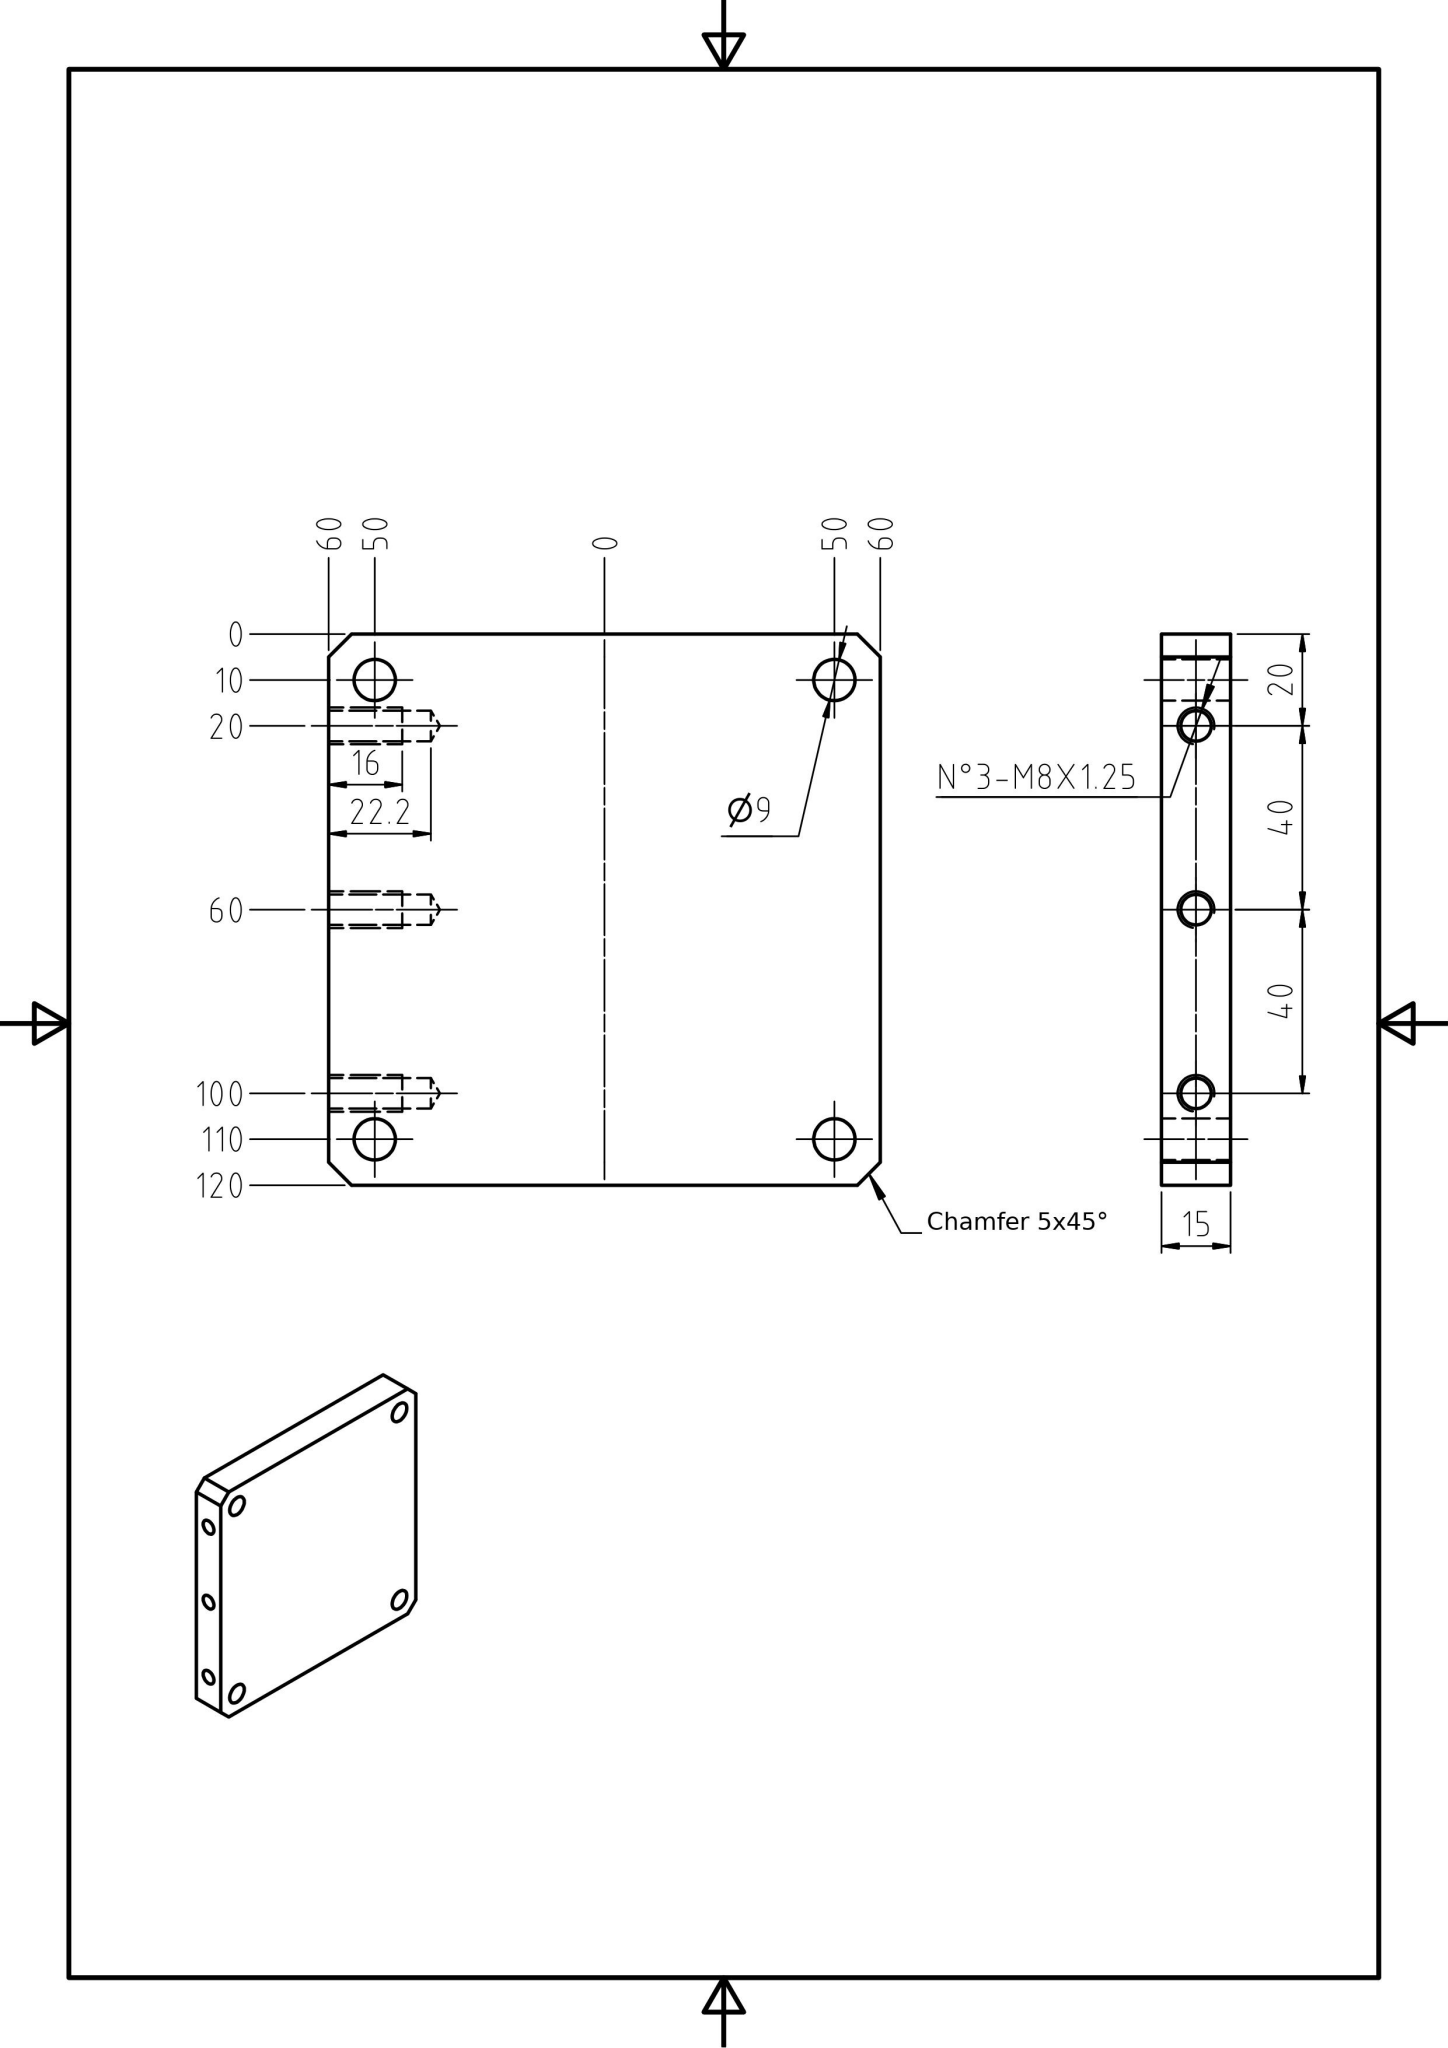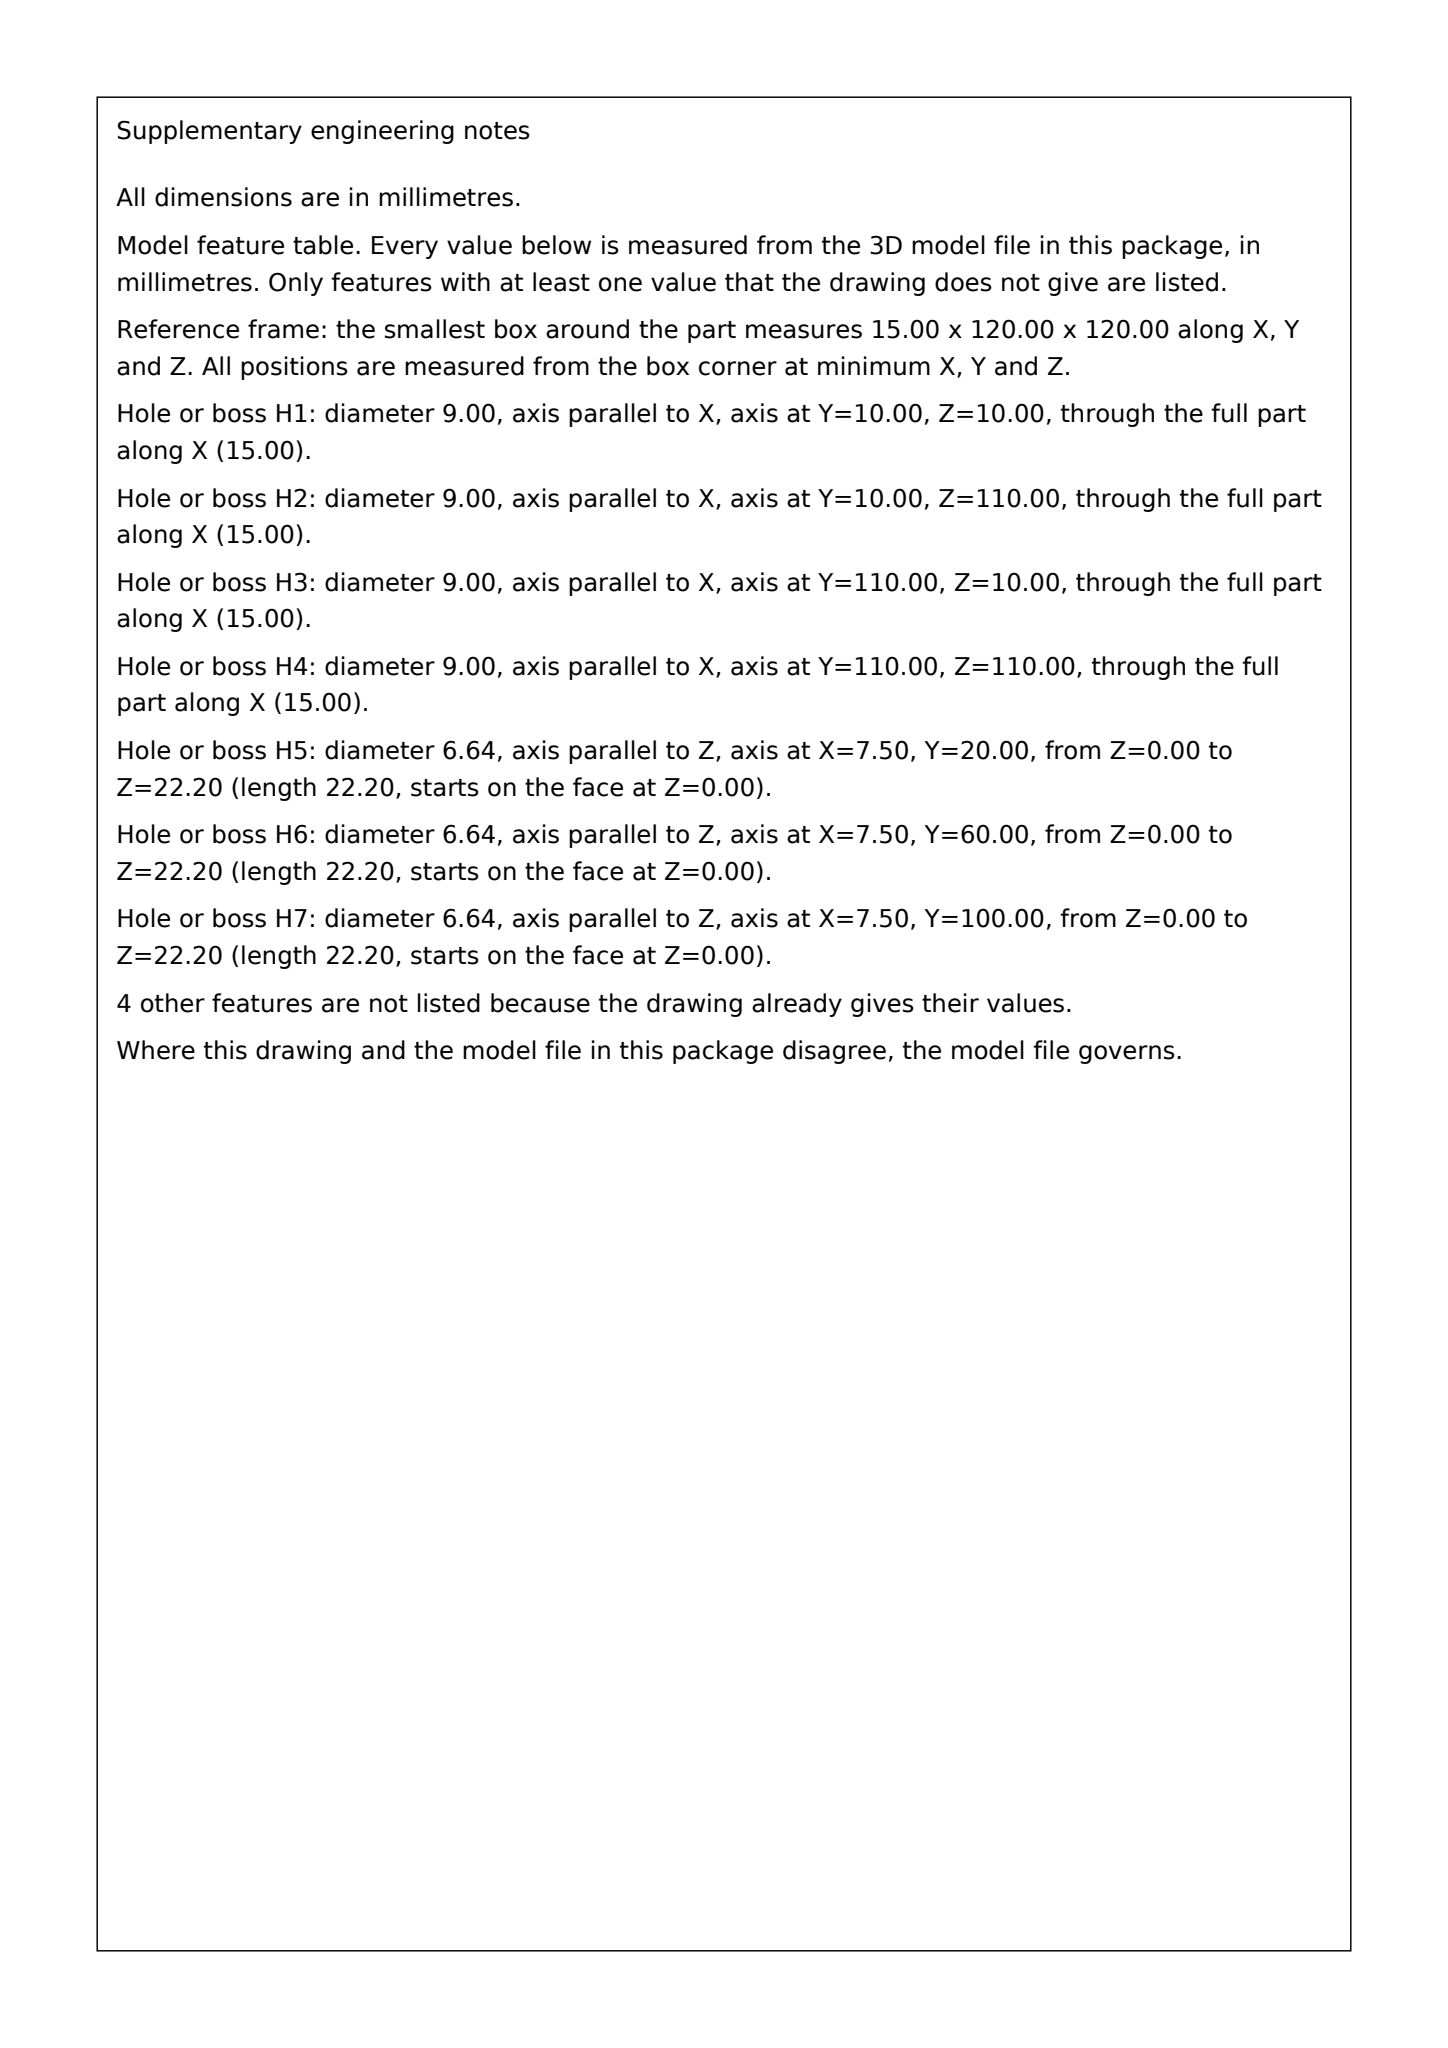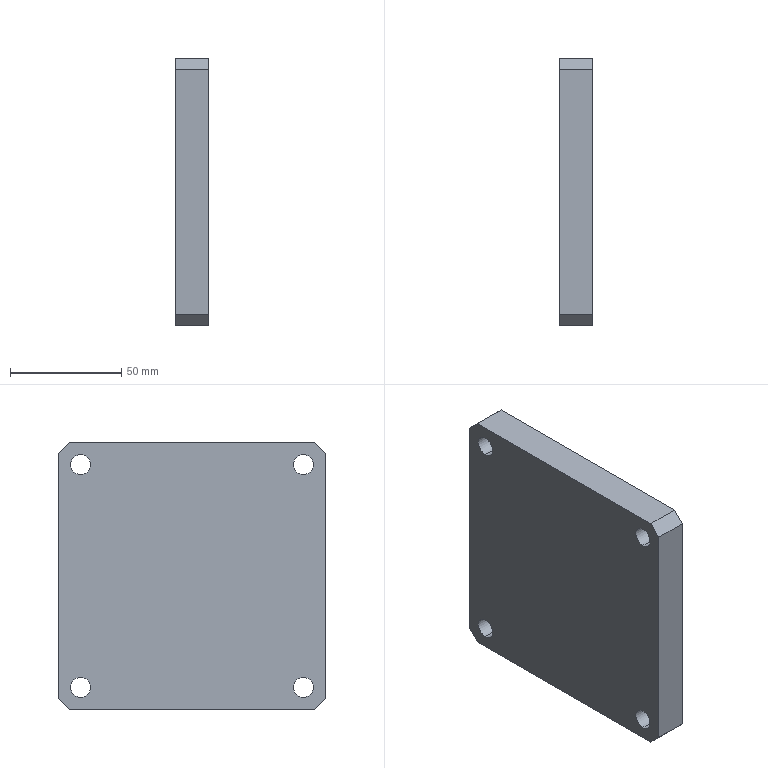Part | SolidWorks | mm | 1 solid | 30 faces | box 15 x 120 x 120 mm | volume 209053 mm3 | cylinder 14 | plane 10 | cone 6 | commonest cylinder face diameters 9 x8 6.647 x6